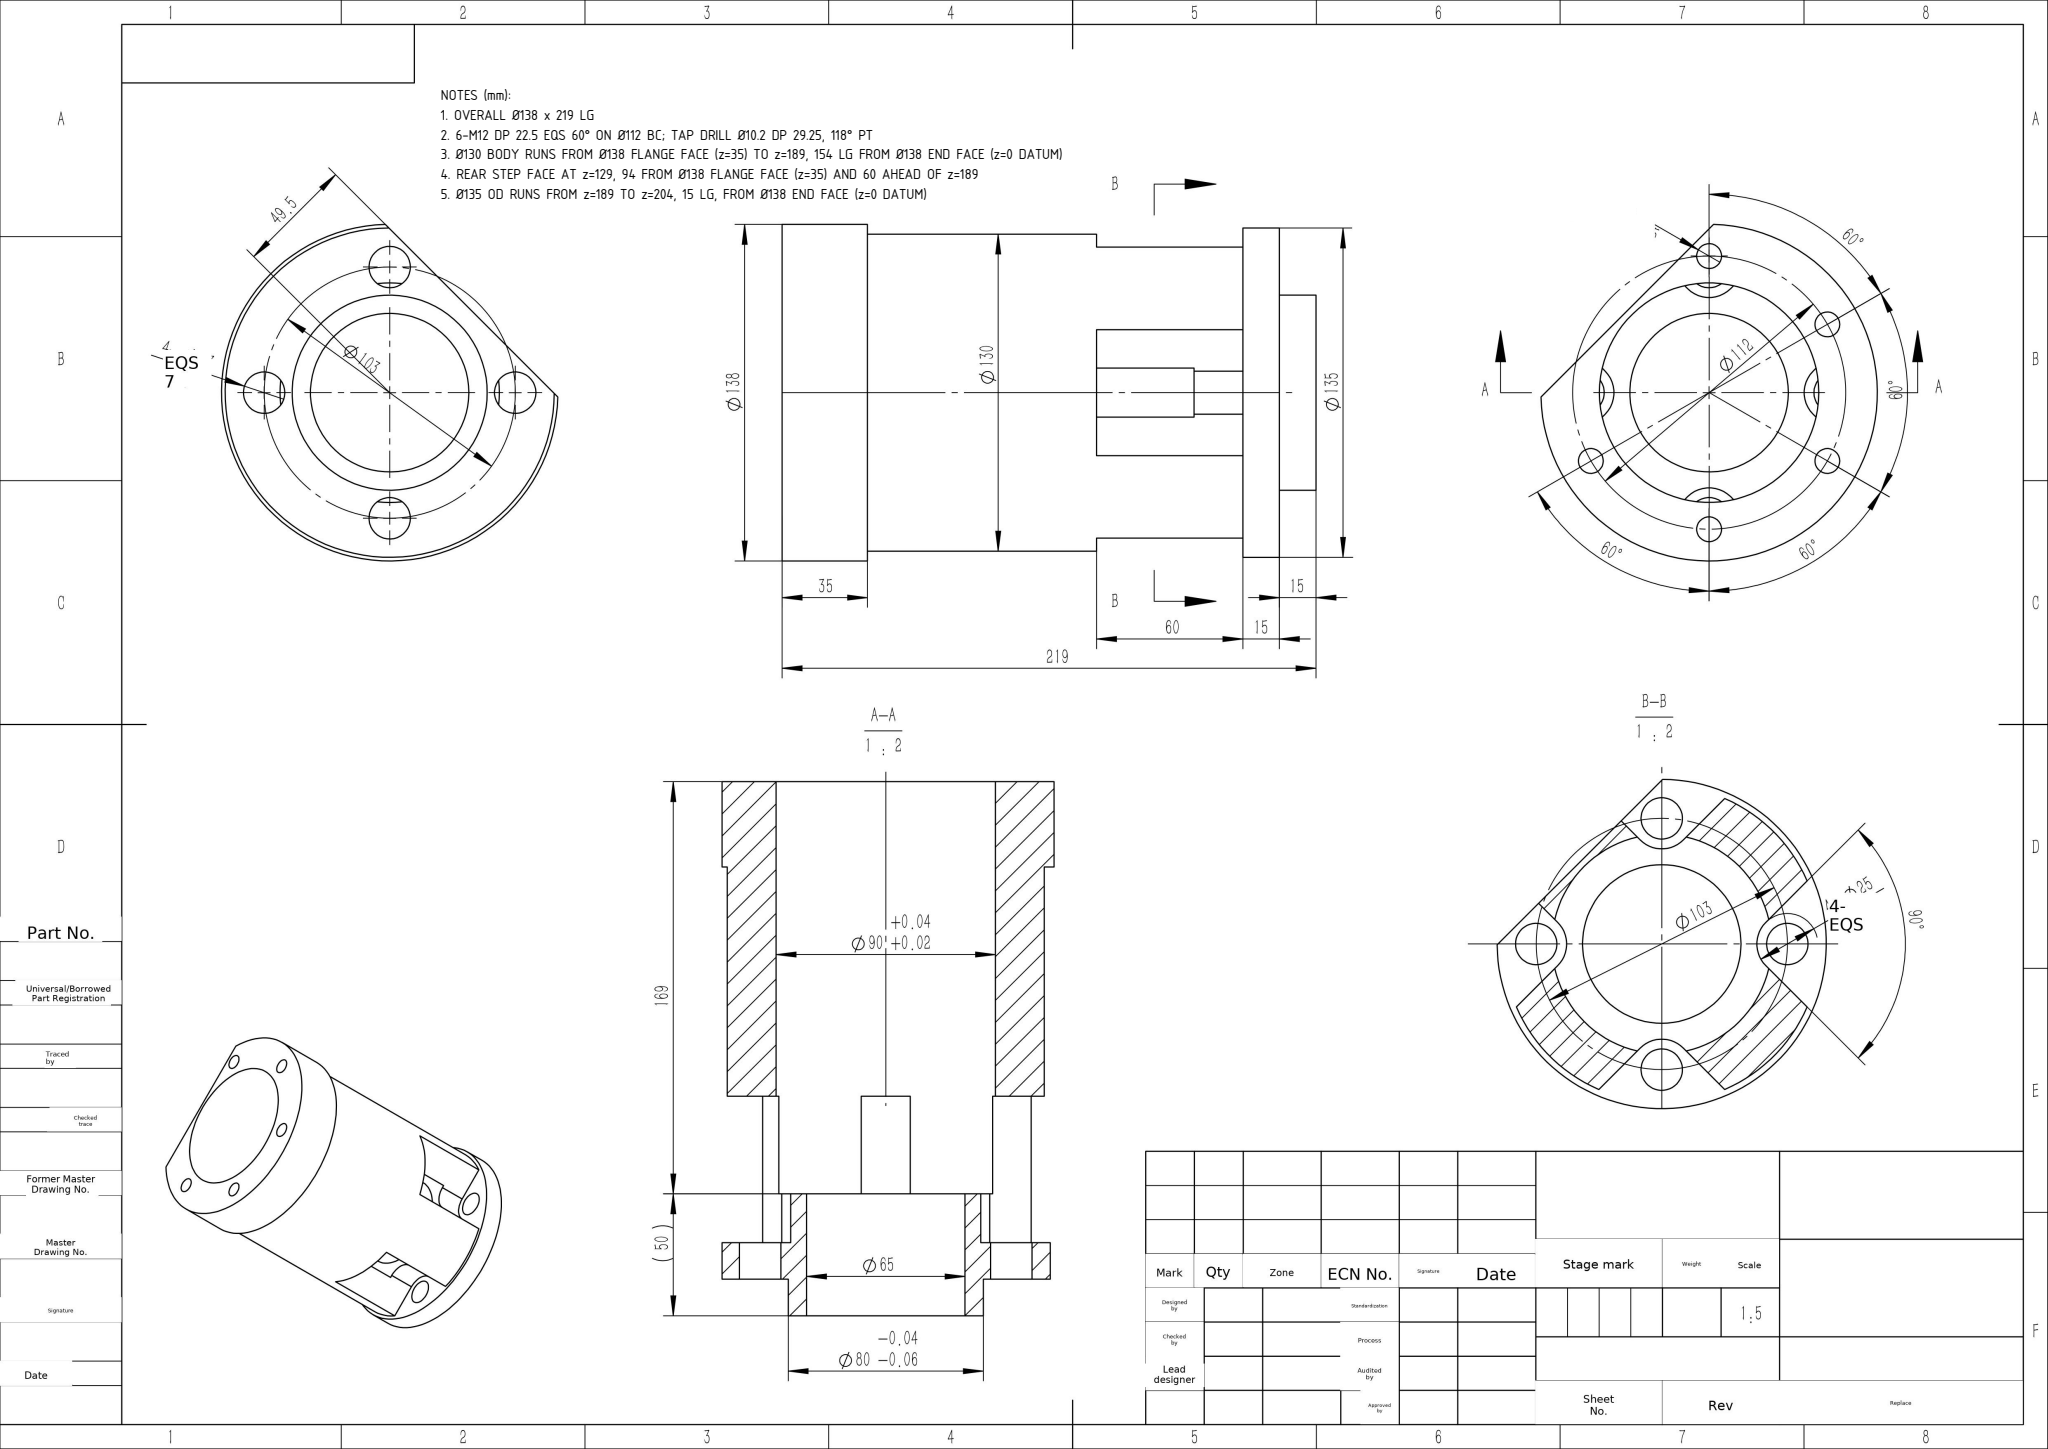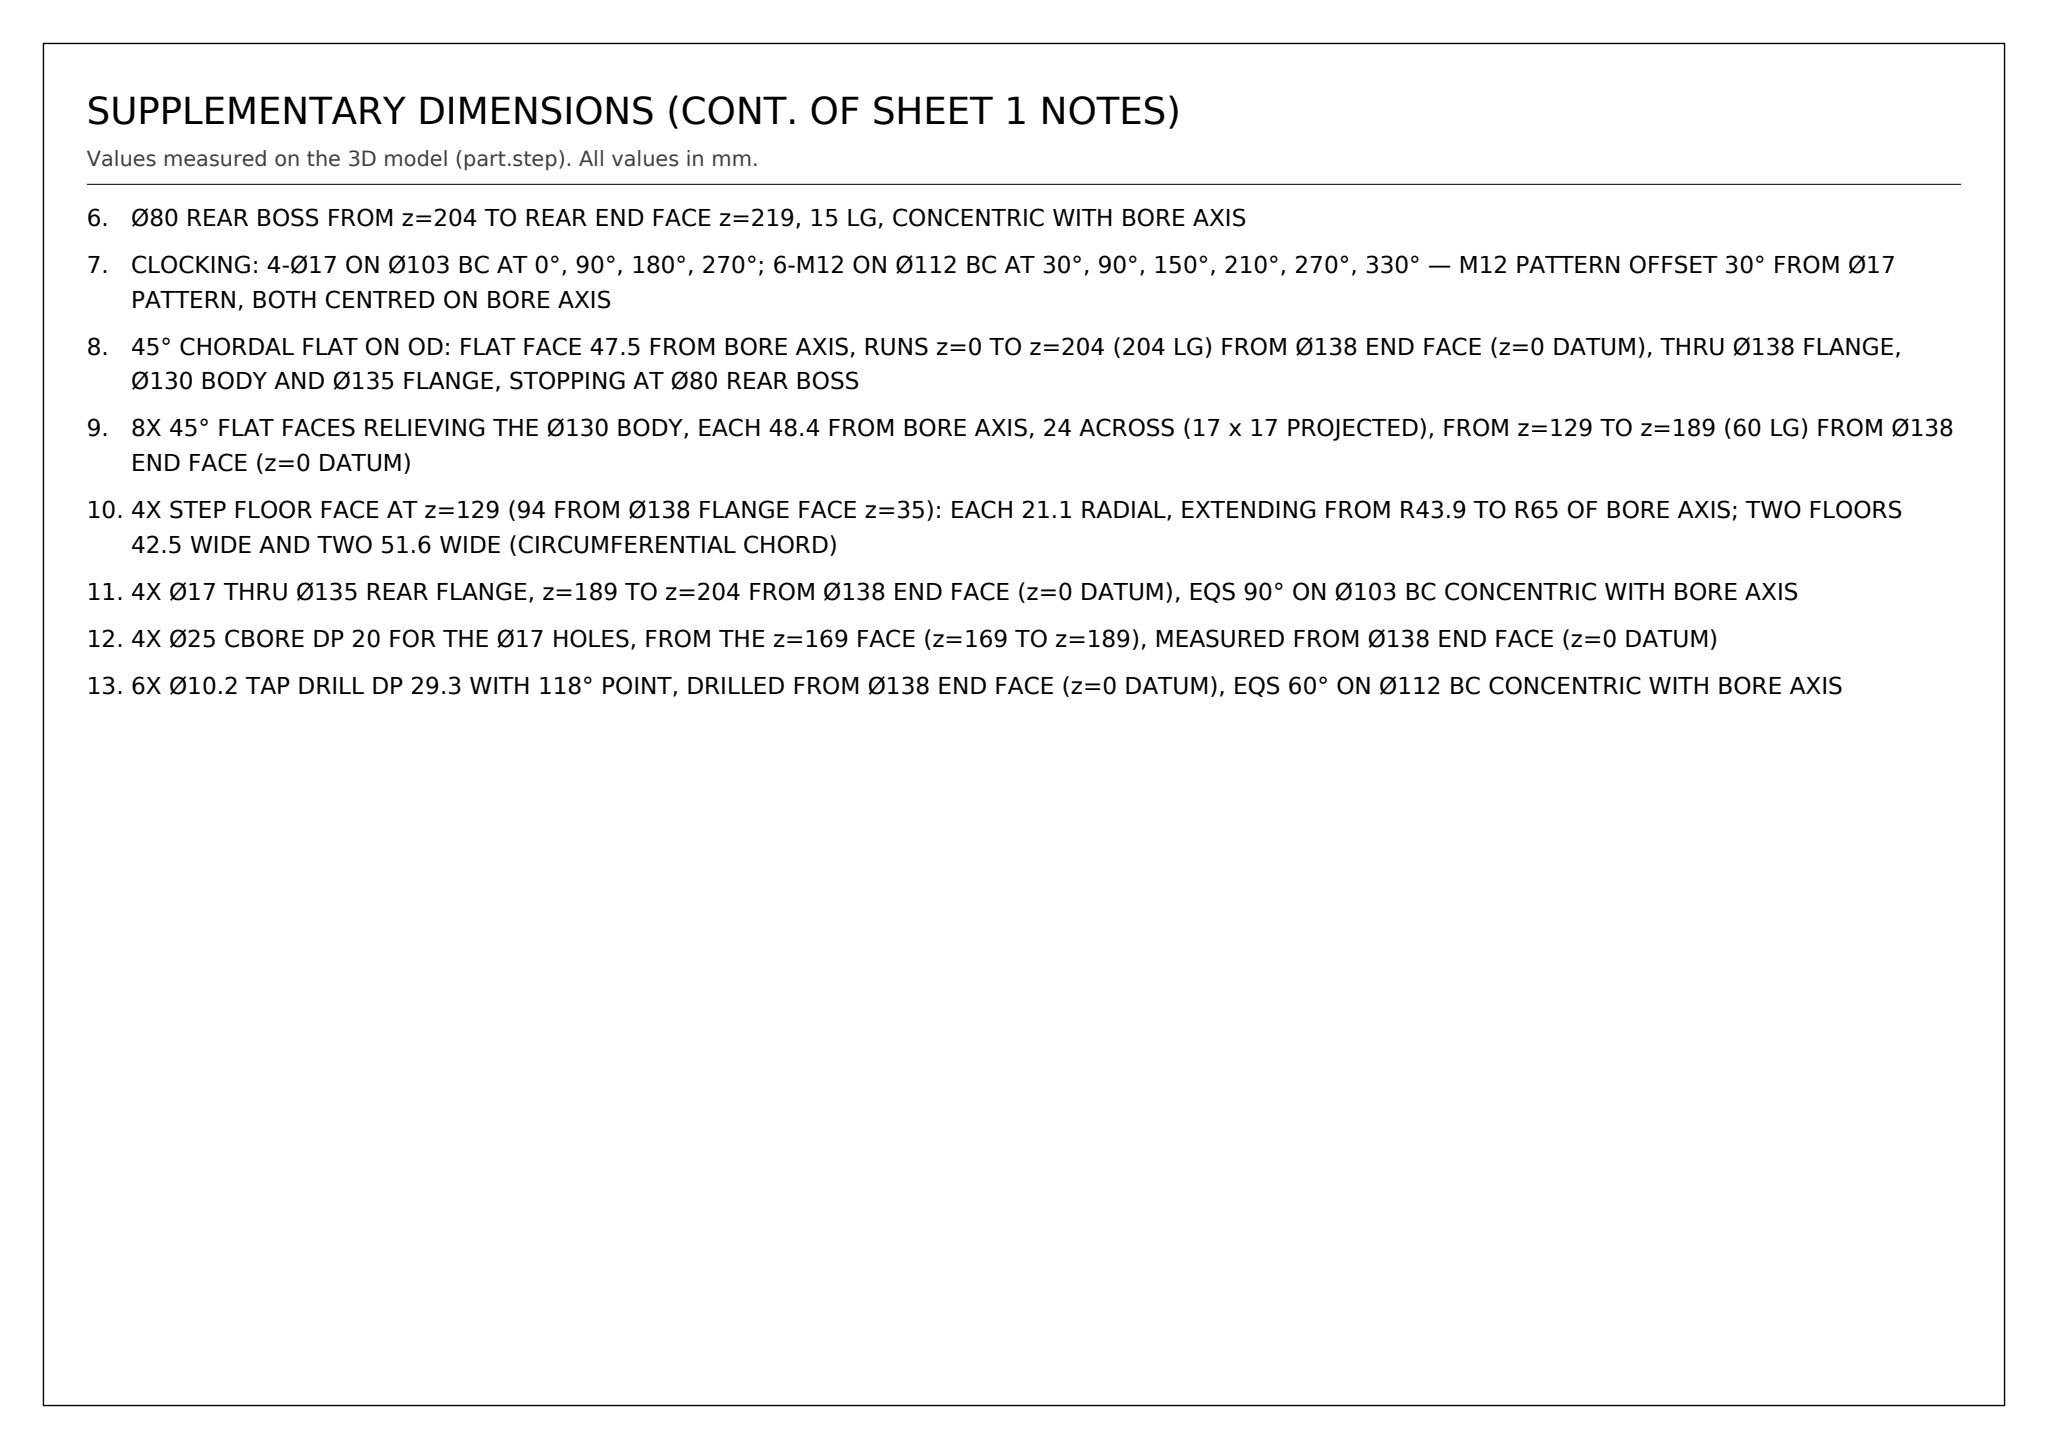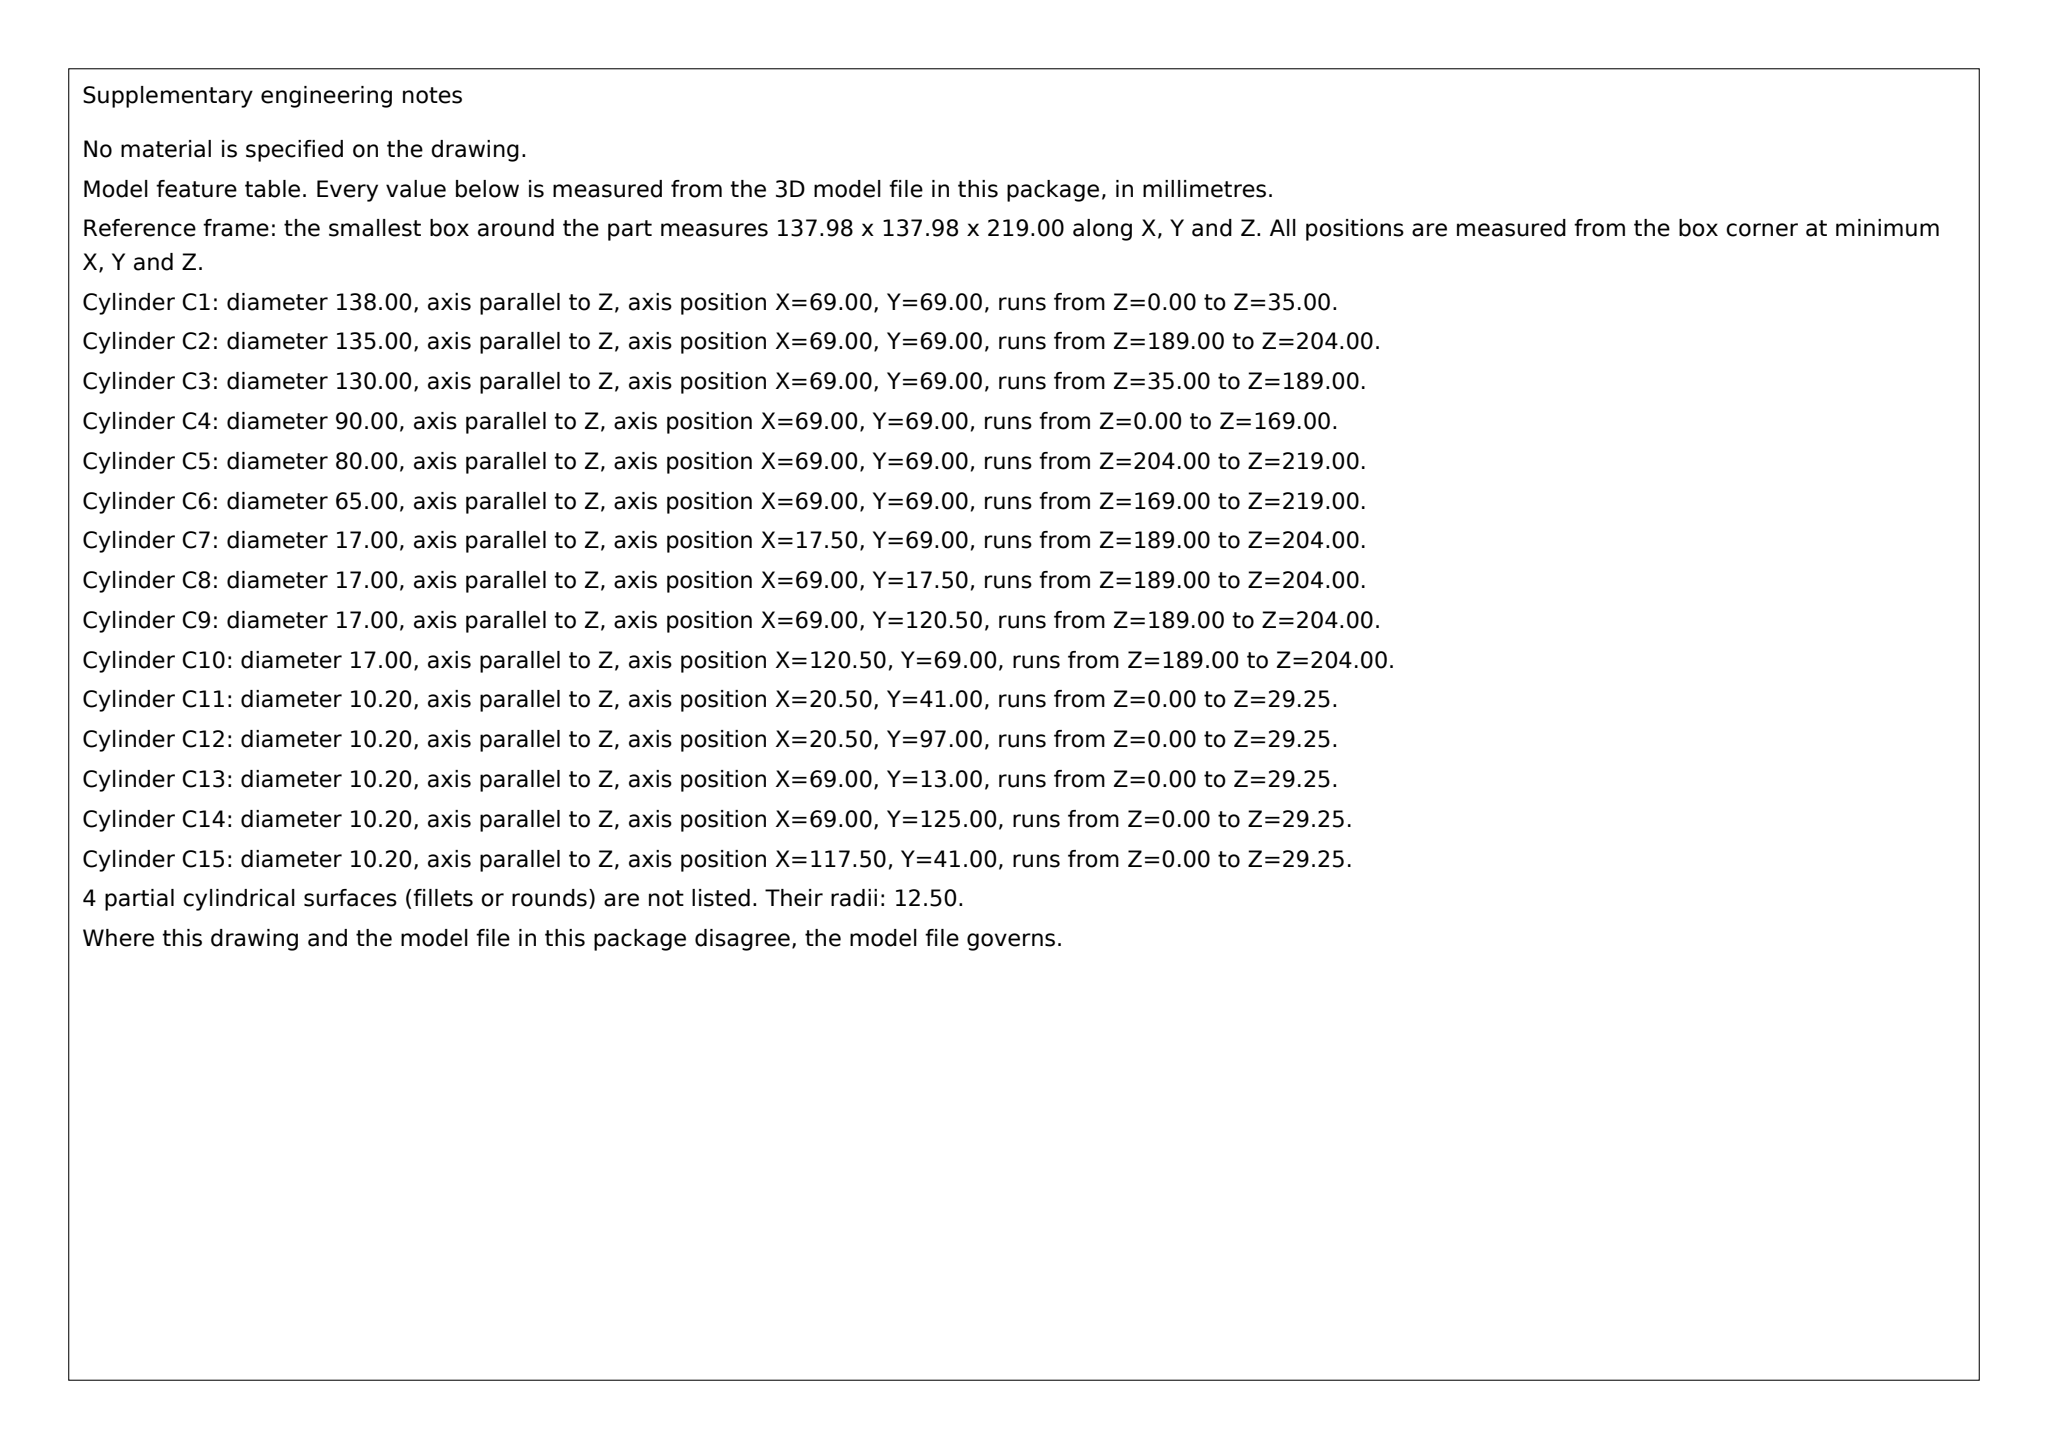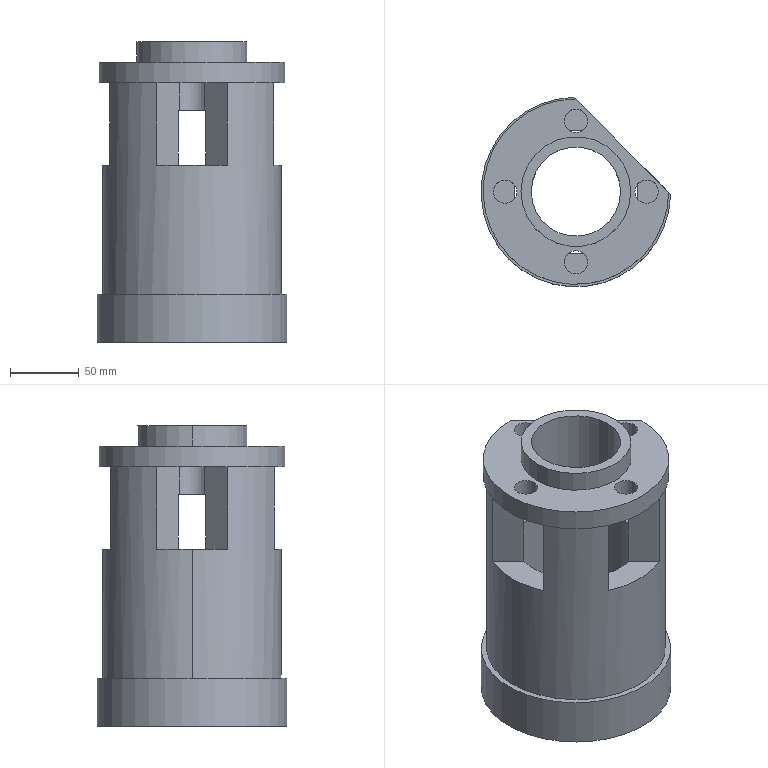Part | SolidWorks | mm | 1 solid | 63 faces | box 137.98 x 137.98 x 219 mm | volume 1189158 mm3 | cylinder 34 | plane 19 | cone 10 | commonest cylinder face diameters 10.2 x10 17 x8 25 x5 130 x3 80 x2 65 x2 90 x2 135 x1
Drawing notes:
OVERALL Ø138 x 219 LG | from the solid: bbox 137.976x137.976x219; Ø138 z-cyl L35, Ø130 L154, Ø135 L15
6-M12 DP 22.5 EQS 60° ON Ø112 BC; TAP DRILL Ø10.2 DP 29.25, 118° PT | from the solid: Ø10.2 z-cyl L29.25 at r=56 from axis (69,69) → Ø112 BC, 6 places; 118° cone ref dia 10.2; eff thd depth 22.5 per sheet note
Ø130 BODY RUNS FROM Ø138 FLANGE FACE (z=35) TO z=189, 154 LG FROM Ø138 END FACE (z=0 DATUM) | from the solid: cylinder dia 130 len 154; axis planes z=35, z=189
REAR STEP FACE AT z=129, 94 FROM Ø138 FLANGE FACE (z=35) AND 60 AHEAD OF z=189 | from the solid: axis_planes z=129 (4 faces); cylinder Ø130 z-axis length 94; cylinder Ø130 length 154 ending z=189
Ø135 OD RUNS FROM z=189 TO z=204, 15 LG, FROM Ø138 END FACE (z=0 DATUM) | from the solid: cylinders: convex arc dia 135, axis z at (69,69), from 189 to 204 (269°)
Ø80 REAR BOSS FROM z=204 TO REAR END FACE z=219, 15 LG, CONCENTRIC WITH BORE AXIS | from the solid: cylinders: boss/shaft dia 80, axis z at (69,69), from 204 to 219 (360°)
CLOCKING: 4-Ø17 ON Ø103 BC AT 0°, 90°, 180°, 270°; 6-M12 ON Ø112 BC AT 30°, 90°, 150°, 210°, 270°, 330° — M12 PATTERN OFFSET 30° FROM Ø17 PATTERN, BOTH CENTRED ON BORE AXIS | from the solid: Ø17 hole centres (120.5,69),(69,120.5),(17.5,69),(69,17.5) at R51.5; Ø10.2 tap-drill centres (117.5,41),(20.5,41),(20.5,97),(69,125),(69,13) at R56 about axis (69,69)
45° CHORDAL FLAT ON OD: FLAT FACE 47.5 FROM BORE AXIS, RUNS z=0 TO z=204 (204 LG) FROM Ø138 END FACE (z=0 DATUM), THRU Ø138 FLANGE, Ø130 BODY AND Ø135 FLANGE, STOPPING AT Ø80 REAR BOSS | from the solid: inclined_planes: angle [45,45,90], bbox_from [67.2,67.2,0.0], size [70.8,70.8,204.0] (offset from axis at x=y=69 computes 47.5)
8X 45° FLAT FACES RELIEVING THE Ø130 BODY, EACH 48.4 FROM BORE AXIS, 24 ACROSS (17 x 17 PROJECTED), FROM z=129 TO z=189 (60 LG) FROM Ø138 END FACE (z=0 DATUM) | from the solid: inclined_planes: 45° faces bbox_from [111.7,43.2,129], [43.2,111.7,129], [43.2,9.4,129], [77.8,9.4,129], [9.4,43.2,129], [9.4,77.8,129] size [17,17,60]; two further 45° faces size [7.8,7.8,60]
4X STEP FLOOR FACE AT z=129 (94 FROM Ø138 FLANGE FACE z=35): EACH 21.1 RADIAL, EXTENDING FROM R43.9 TO R65 OF BORE AXIS; TWO FLOORS 42.5 WIDE AND TWO 51.6 WIDE (CIRCUMFERENTIAL CHORD) | from the solid: axis_planes z=129: extents x[112.9,134.0] y[43.2,85.7] area 586 (x2) and x[4.0,25.1] y[43.2,94.8] area 737 (x2)
4X Ø17 THRU Ø135 REAR FLANGE, z=189 TO z=204 FROM Ø138 END FACE (z=0 DATUM), EQS 90° ON Ø103 BC CONCENTRIC WITH BORE AXIS | from the solid: cylinders hole/bore Ø17 at (120.5,69), (17.5,69), (69,120.5), (69,17.5), from 189.0 to 204.0 (R51.5 = Ø103 BC)
4X Ø25 CBORE DP 20 FOR THE Ø17 HOLES, FROM THE z=169 FACE (z=169 TO z=189), MEASURED FROM Ø138 END FACE (z=0 DATUM) | from the solid: cylinders Ø25 arcs at (120.5,69), (17.5,69), (69,120.5), (69,17.5), from 169.0 to 189.0
6X Ø10.2 TAP DRILL DP 29.3 WITH 118° POINT, DRILLED FROM Ø138 END FACE (z=0 DATUM), EQS 60° ON Ø112 BC CONCENTRIC WITH BORE AXIS | from the solid: cylinders hole/bore Ø10.2 from 0.0 to 29.3 at (117.5,41), (20.5,41), (20.5,97), (69,125), (69,13) (R56 = Ø112 BC); cones 118° ref_dia 10.2 at z=29.3